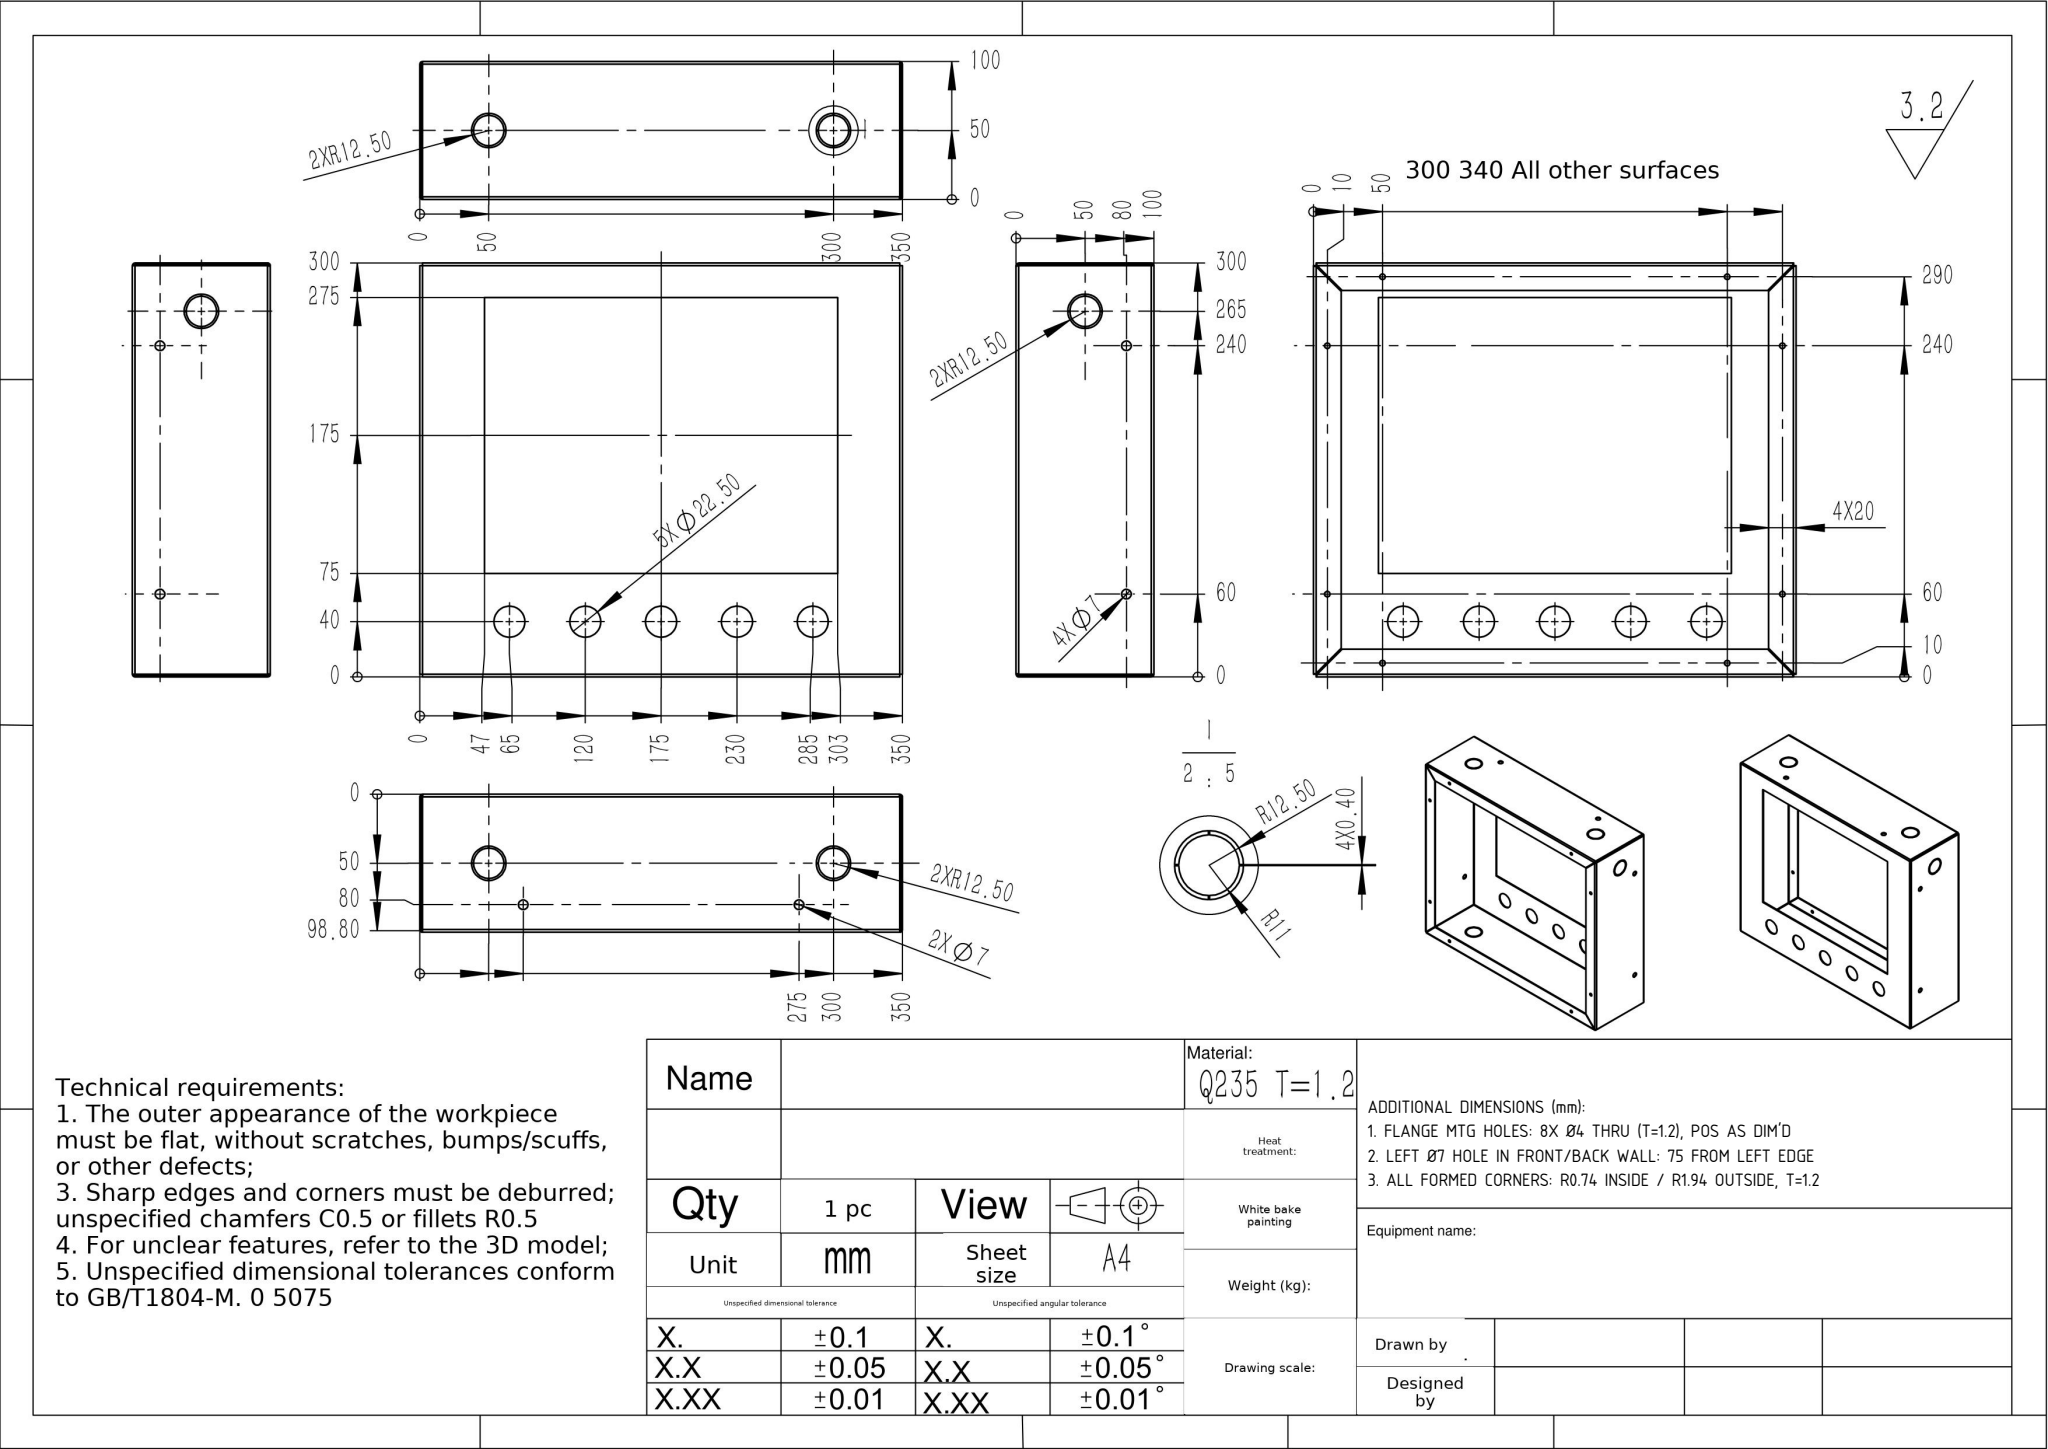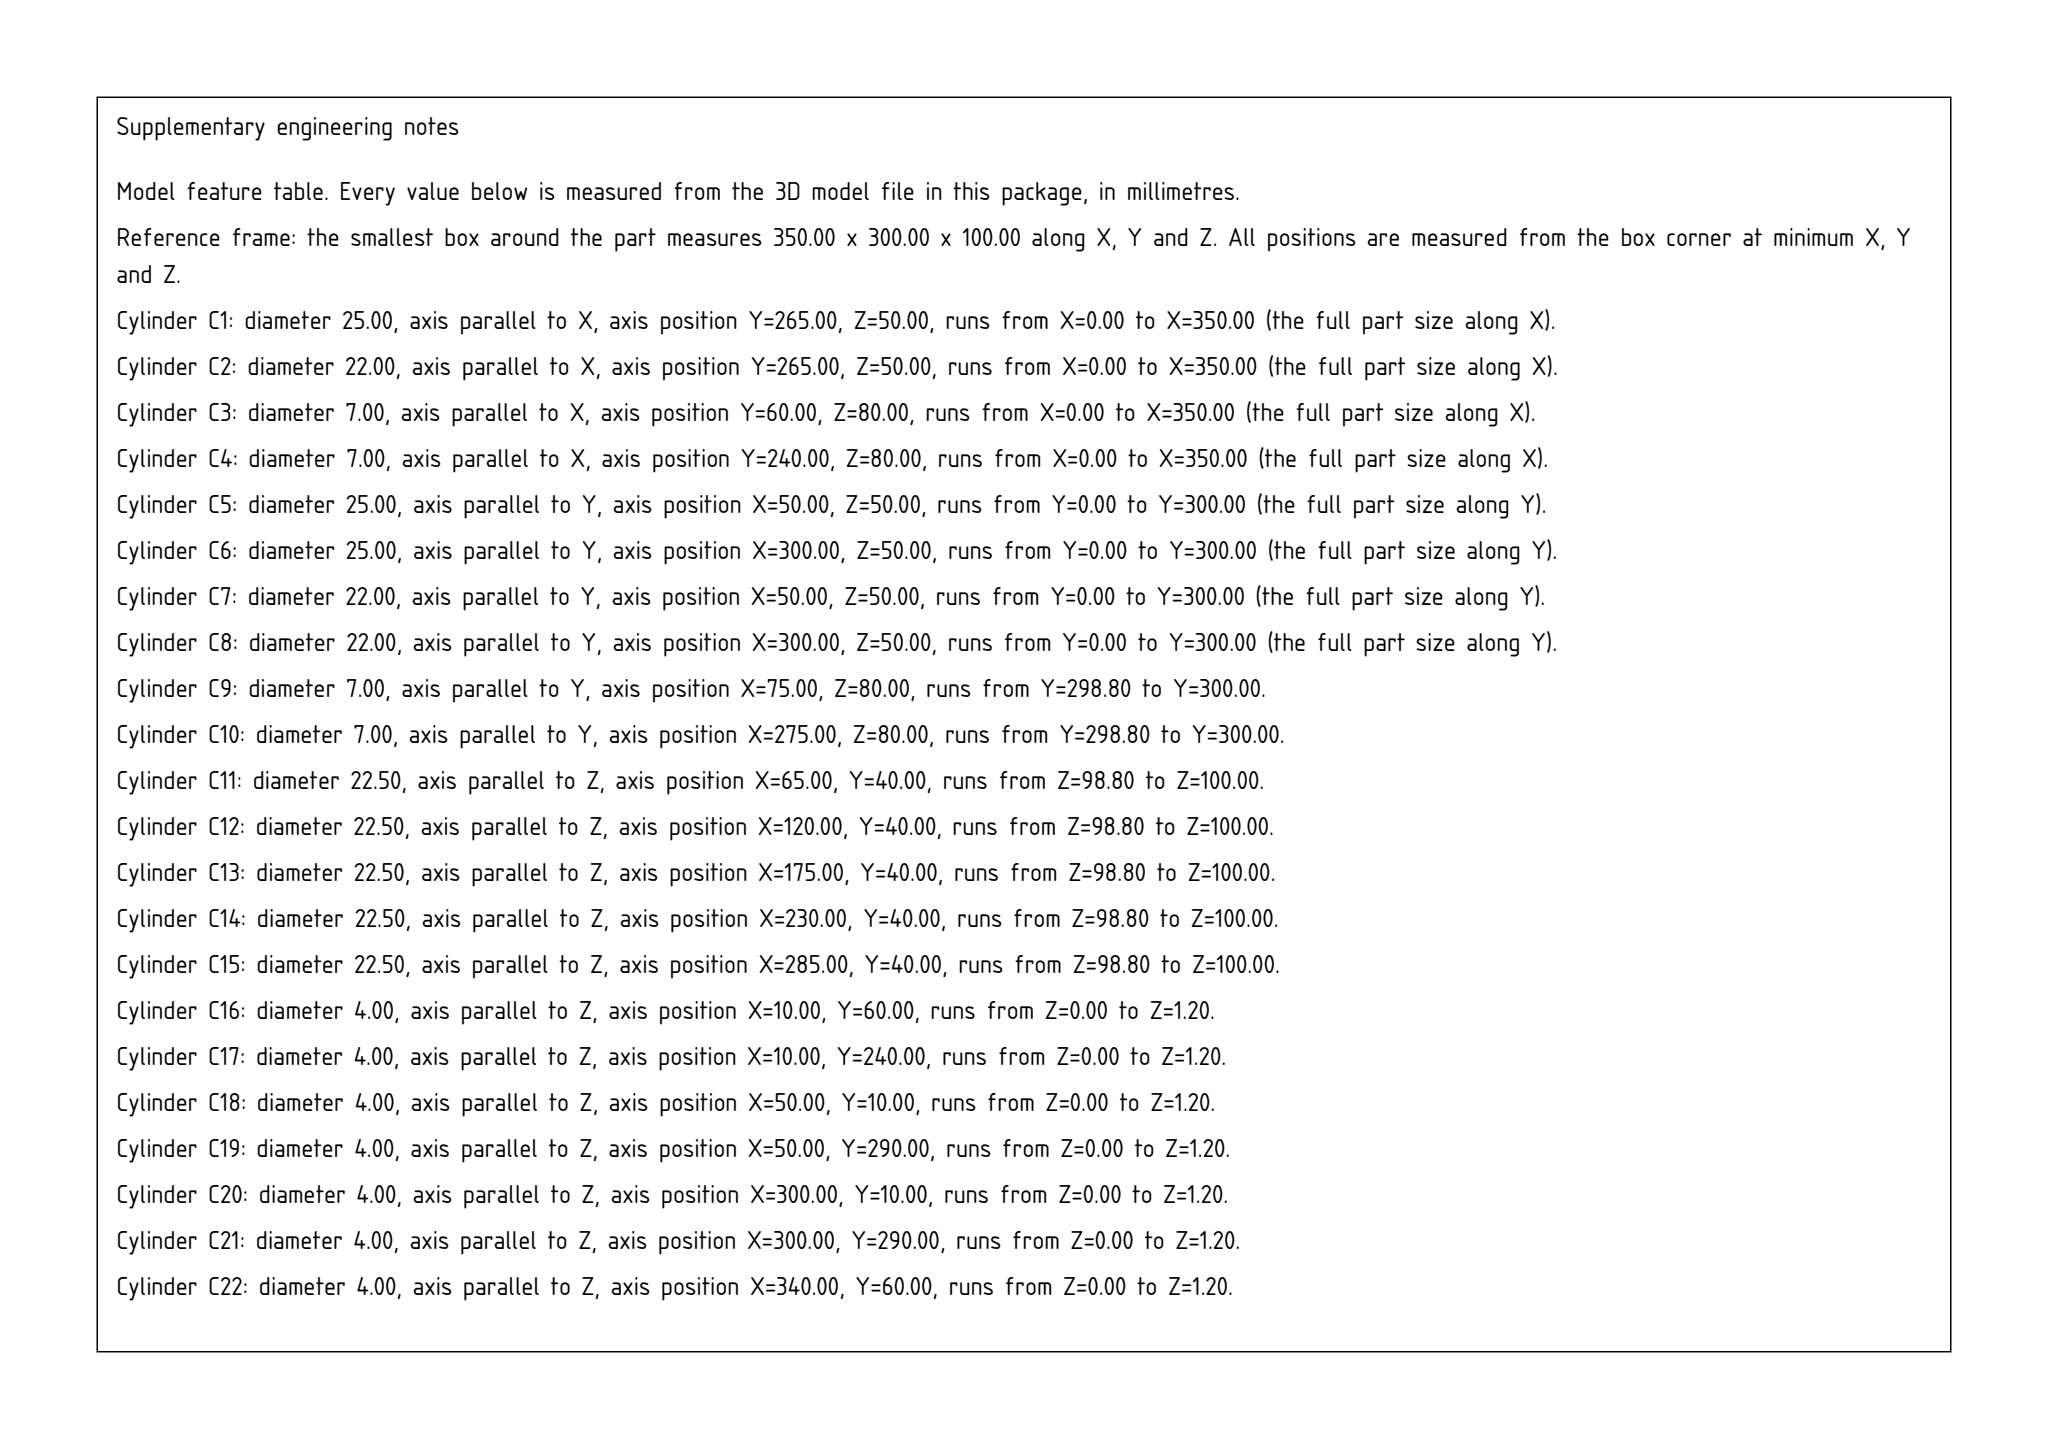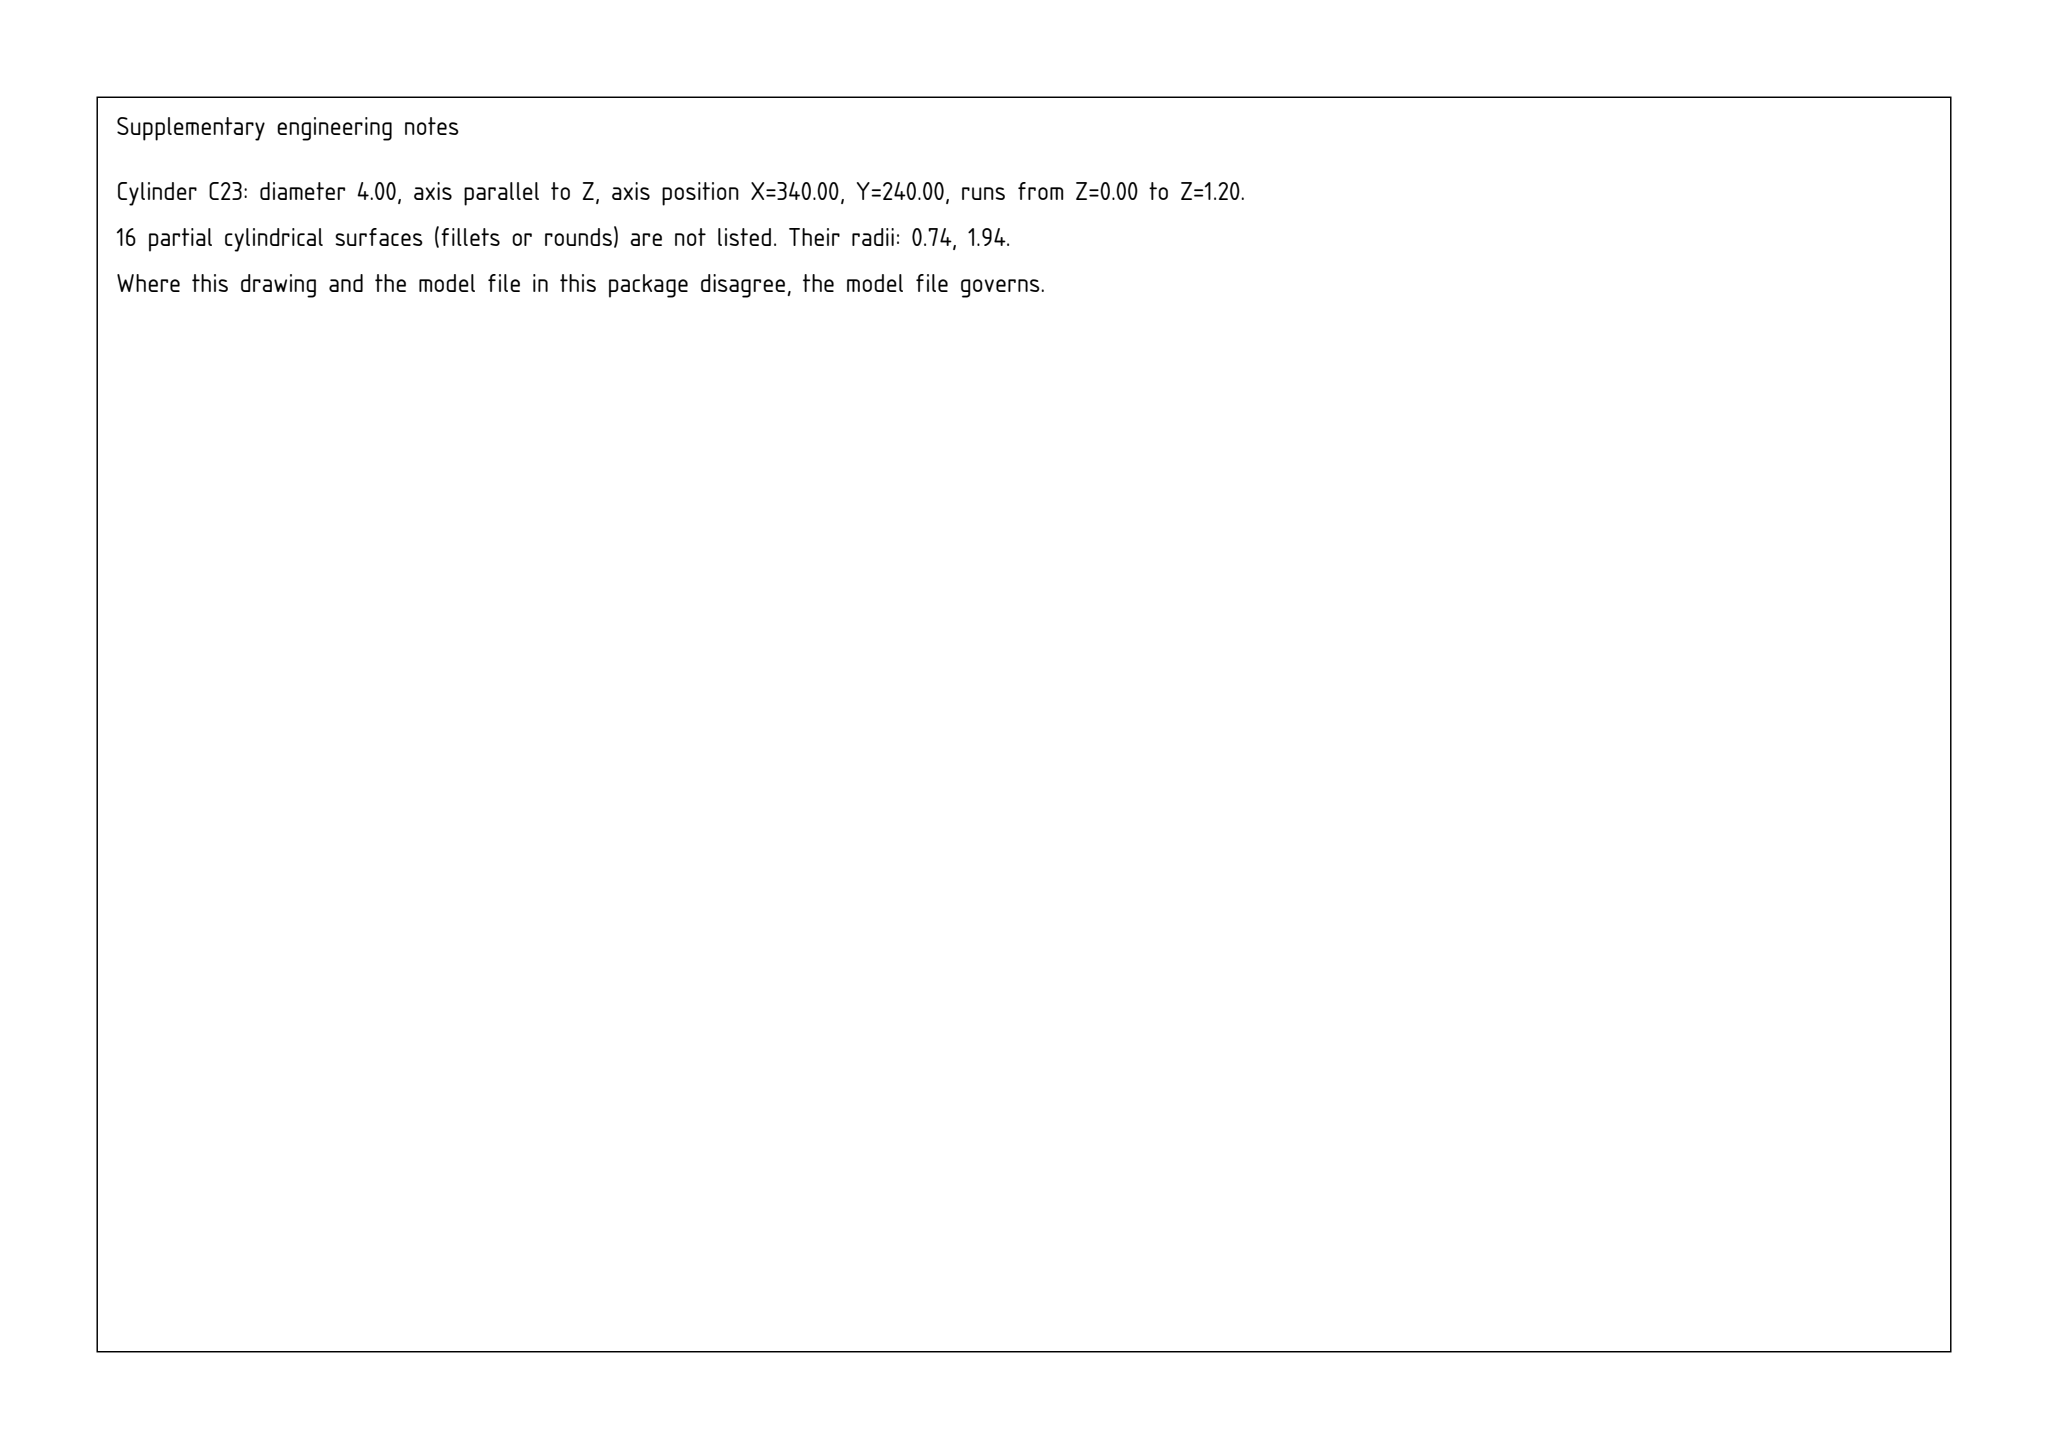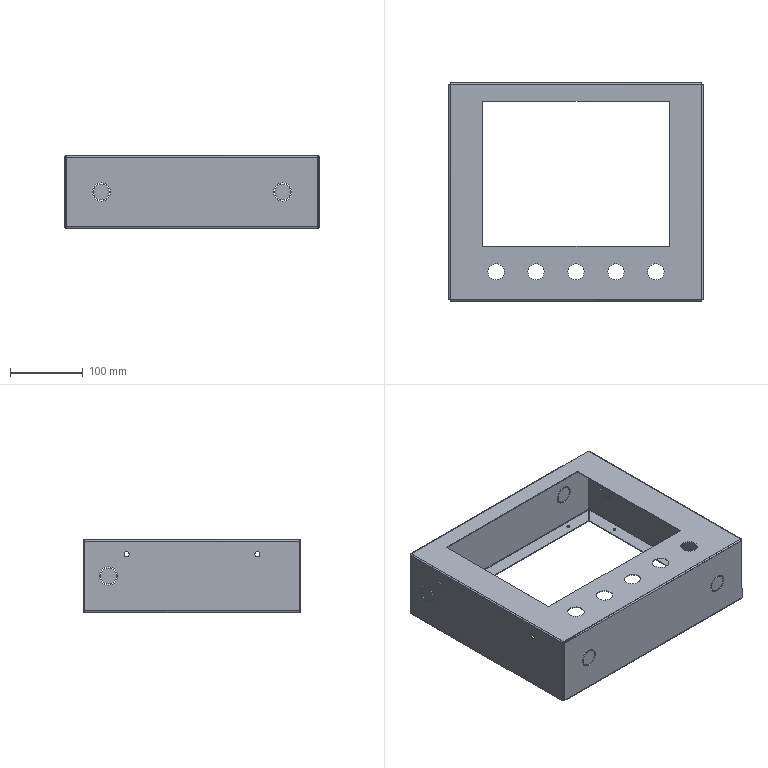Part | SolidWorks | mm | 1 solid | 208 faces | box 350 x 300 x 100 mm | volume 238812 mm3 | cylinder 102 | plane 90 | spline 16 | commonest cylinder face diameters 22 x24 25 x24 4 x16 7 x12 22.5 x10 3.873 x8 1.473 x8